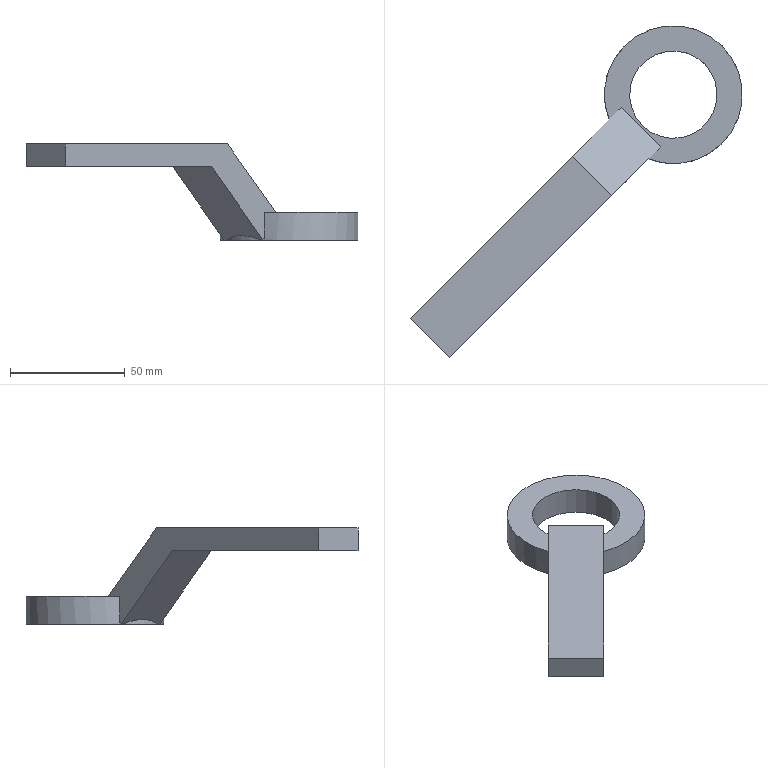Component | NX | WRENCH | 1 solid | 14 faces | box 144.55 x 144.55 x 41.82 mm | volume 56359 mm3 | plane 11 | cylinder 3 | commonest cylinder face diameters 60 x2 38 x1
STEP:
#1=CARTESIAN_POINT('',(0.,0.,0.));
#2=DIRECTION('',(0.,0.,1.));
#3=DIRECTION('',(1.,0.,0.));
#4=AXIS2_PLACEMENT_3D('',#1,#2,#3);
#5=CARTESIAN_POINT('',(53.835,-128.832,-32.615));
#6=VERTEX_POINT('',#5);
#7=CARTESIAN_POINT('',(69.066,-144.064,-32.615));
#8=VERTEX_POINT('',#7);
#9=CARTESIAN_POINT('',(81.249,-116.649,-32.615));
#10=DIRECTION('',(0.,0.,1.));
#11=DIRECTION('',(-0.7071,-0.7071,0.));
#12=AXIS2_PLACEMENT_3D('',#9,#10,#11);
#13=CIRCLE('',#12,30.);
#14=CARTESIAN_POINT('',(81.249,-116.649,-32.615));
#15=DIRECTION('',(0.,0.,1.));
#16=DIRECTION('',(-0.7071,-0.7071,0.));
#17=AXIS2_PLACEMENT_3D('',#14,#15,#16);
#18=CYLINDRICAL_SURFACE('',#17,30.);
#19=CARTESIAN_POINT('',(0.,0.));
#20=DIRECTION('',(1.,0.));
#21=VECTOR('',#20,1.);
#22=LINE('',#19,#21);
#23=(GEOMETRIC_REPRESENTATION_CONTEXT(2)PARAMETRIC_REPRESENTATION_CONTEXT()REPRESENTATION_CONTEXT('',''));
#24=DEFINITIONAL_REPRESENTATION('',(#22),#23);
#25=PCURVE('',#18,#24);
#26=CARTESIAN_POINT('',(81.249,-116.649,-32.615));
#27=DIRECTION('',(0.,0.,-1.));
#28=DIRECTION('',(0.7071,0.7071,0.));
#29=AXIS2_PLACEMENT_3D('',#26,#27,#28);
#30=PLANE('',#29);
#31=CARTESIAN_POINT('',(-30.,0.));
#32=CARTESIAN_POINT('',(-30.,51.962));
#33=CARTESIAN_POINT('',(15.,25.981));
#34=CARTESIAN_POINT('',(60.,0.));
#35=CARTESIAN_POINT('',(15.,-25.981));
#36=CARTESIAN_POINT('',(-30.,-51.962));
#37=CARTESIAN_POINT('',(-30.,0.));
#38=(BOUNDED_CURVE()B_SPLINE_CURVE(2,(#31,#32,#33,#34,#35,#36,#37),.UNSPECIFIED.,.T.,.F.)B_SPLINE_CURVE_WITH_KNOTS((1,2,2,2,2,1),(-2.094,0.,2.094,4.189,6.283,8.378),.UNSPECIFIED.)CURVE()GEOMETRIC_REPRESENTATION_ITEM()RATIONAL_B_SPLINE_CURVE((1.,0.5,1.,0.5,1.,0.5,1.))REPRESENTATION_ITEM(''));
#39=(GEOMETRIC_REPRESENTATION_CONTEXT(2)PARAMETRIC_REPRESENTATION_CONTEXT()REPRESENTATION_CONTEXT('',''));
#40=DEFINITIONAL_REPRESENTATION('',(#38),#39);
#41=PCURVE('',#30,#40);
#42=SURFACE_CURVE('',#13,(#25,#41),.PCURVE_S1.);
#43=EDGE_CURVE('',#6,#8,#42,.T.);
#44=ORIENTED_EDGE('',*,*,#43,.T.);
#45=CARTESIAN_POINT('',(81.249,-116.649,-60.615));
#46=DIRECTION('',(-0.5,-0.5,-0.7071));
#47=DIRECTION('',(-0.5,-0.5,0.7071));
#48=AXIS2_PLACEMENT_3D('',#45,#46,#47);
#49=ELLIPSE('',#48,42.426,30.);
#50=CARTESIAN_POINT('',(6.65,-0.));
#51=CARTESIAN_POINT('',(6.639,0.1198));
#52=CARTESIAN_POINT('',(6.617,0.3491));
#53=CARTESIAN_POINT('',(6.584,0.6615));
#54=CARTESIAN_POINT('',(6.55,0.9419));
#55=CARTESIAN_POINT('',(6.517,1.19));
#56=CARTESIAN_POINT('',(6.483,1.406));
#57=CARTESIAN_POINT('',(6.45,1.589));
#58=CARTESIAN_POINT('',(6.417,1.738));
#59=CARTESIAN_POINT('',(6.383,1.855));
#60=CARTESIAN_POINT('',(6.35,1.939));
#61=CARTESIAN_POINT('',(6.317,1.989));
#62=CARTESIAN_POINT('',(6.283,2.006));
#63=CARTESIAN_POINT('',(6.25,1.989));
#64=CARTESIAN_POINT('',(6.216,1.939));
#65=CARTESIAN_POINT('',(6.183,1.855));
#66=CARTESIAN_POINT('',(6.15,1.738));
#67=CARTESIAN_POINT('',(6.116,1.589));
#68=CARTESIAN_POINT('',(6.083,1.406));
#69=CARTESIAN_POINT('',(6.05,1.19));
#70=CARTESIAN_POINT('',(6.016,0.9419));
#71=CARTESIAN_POINT('',(5.983,0.6615));
#72=CARTESIAN_POINT('',(5.949,0.3491));
#73=CARTESIAN_POINT('',(5.927,0.1198));
#74=CARTESIAN_POINT('',(5.916,-0.));
#75=B_SPLINE_CURVE_WITH_KNOTS('',3,(#50,#51,#52,#53,#54,#55,#56,#57,#58,#59,#60,#61,#62,#63,#64,#65,#66,#67,#68,#69,#70,#71,#72,#73,#74),.UNSPECIFIED.,.F.,.F.,(4,1,1,1,1,1,1,1,1,1,1,1,1,1,1,1,1,1,1,1,1,1,4),(5.916,5.949,5.983,6.016,6.05,6.083,6.116,6.15,6.183,6.216,6.25,6.283,6.317,6.35,6.383,6.417,6.45,6.483,6.517,6.55,6.584,6.617,6.65),.QUASI_UNIFORM_KNOTS.);
#76=(GEOMETRIC_REPRESENTATION_CONTEXT(2)PARAMETRIC_REPRESENTATION_CONTEXT()REPRESENTATION_CONTEXT('',''));
#77=DEFINITIONAL_REPRESENTATION('',(#75),#76);
#78=PCURVE('',#18,#77);
#79=CARTESIAN_POINT('',(52.965,-127.963,-32.615));
#80=DIRECTION('',(0.5,0.5,0.7071));
#81=DIRECTION('',(-0.5,-0.5,0.7071));
#82=AXIS2_PLACEMENT_3D('',#79,#80,#81);
#83=PLANE('',#82);
#84=CARTESIAN_POINT('',(2.828,12.));
#85=CARTESIAN_POINT('',(2.828,-39.962));
#86=CARTESIAN_POINT('',(-60.811,-13.981));
#87=CARTESIAN_POINT('',(-124.451,12.));
#88=CARTESIAN_POINT('',(-60.811,37.981));
#89=CARTESIAN_POINT('',(2.828,63.962));
#90=CARTESIAN_POINT('',(2.828,12.));
#91=(BOUNDED_CURVE()B_SPLINE_CURVE(2,(#84,#85,#86,#87,#88,#89,#90),.UNSPECIFIED.,.T.,.F.)B_SPLINE_CURVE_WITH_KNOTS((1,2,2,2,2,1),(-2.094,0.,2.094,4.189,6.283,8.378),.UNSPECIFIED.)CURVE()GEOMETRIC_REPRESENTATION_ITEM()RATIONAL_B_SPLINE_CURVE((1.,0.5,1.,0.5,1.,0.5,1.))REPRESENTATION_ITEM(''));
#92=(GEOMETRIC_REPRESENTATION_CONTEXT(2)PARAMETRIC_REPRESENTATION_CONTEXT()REPRESENTATION_CONTEXT('',''));
#93=DEFINITIONAL_REPRESENTATION('',(#91),#92);
#94=PCURVE('',#83,#93);
#95=SURFACE_CURVE('',#49,(#78,#94),.PCURVE_S1.);
#96=EDGE_CURVE('',#8,#6,#95,.T.);
#97=ORIENTED_EDGE('',*,*,#96,.T.);
#98=EDGE_LOOP('',(#44,#97));
#99=FACE_BOUND('',#98,.T.);
#100=ADVANCED_FACE('',(#99),#18,.T.);
#101=CARTESIAN_POINT('',(58.494,-122.434,-20.615));
#102=VERTEX_POINT('',#101);
#103=CARTESIAN_POINT('',(53.322,-127.606,-20.615));
#104=VERTEX_POINT('',#103);
#105=CARTESIAN_POINT('',(72.764,-108.164,-20.615));
#106=DIRECTION('',(-0.7071,-0.7071,0.));
#107=VECTOR('',#106,1.);
#108=LINE('',#105,#107);
#109=CARTESIAN_POINT('',(81.249,-116.649,-20.615));
#110=DIRECTION('',(0.,0.,1.));
#111=DIRECTION('',(-0.7071,-0.7071,0.));
#112=AXIS2_PLACEMENT_3D('',#109,#110,#111);
#113=PLANE('',#112);
#114=CARTESIAN_POINT('',(-0.,-12.));
#115=DIRECTION('',(1.,0.));
#116=VECTOR('',#115,1.);
#117=LINE('',#114,#116);
#118=(GEOMETRIC_REPRESENTATION_CONTEXT(2)PARAMETRIC_REPRESENTATION_CONTEXT()REPRESENTATION_CONTEXT('',''));
#119=DEFINITIONAL_REPRESENTATION('',(#117),#118);
#120=PCURVE('',#113,#119);
#121=CARTESIAN_POINT('',(72.764,-108.164,-32.615));
#122=DIRECTION('',(-0.7071,0.7071,0.));
#123=DIRECTION('',(0.,0.,-1.));
#124=AXIS2_PLACEMENT_3D('',#121,#122,#123);
#125=PLANE('',#124);
#126=CARTESIAN_POINT('',(-12.,0.));
#127=DIRECTION('',(0.,1.));
#128=VECTOR('',#127,1.);
#129=LINE('',#126,#128);
#130=(GEOMETRIC_REPRESENTATION_CONTEXT(2)PARAMETRIC_REPRESENTATION_CONTEXT()REPRESENTATION_CONTEXT('',''));
#131=DEFINITIONAL_REPRESENTATION('',(#129),#130);
#132=PCURVE('',#125,#131);
#133=SURFACE_CURVE('',#108,(#120,#132),.PCURVE_S1.);
#134=EDGE_CURVE('',#102,#104,#133,.T.);
#135=ORIENTED_EDGE('',*,*,#134,.F.);
#136=CARTESIAN_POINT('',(75.465,-139.404,-20.615));
#137=VERTEX_POINT('',#136);
#138=CARTESIAN_POINT('',(58.494,-122.434,-20.615));
#139=DIRECTION('',(0.7071,-0.7071,0.));
#140=VECTOR('',#139,1.);
#141=LINE('',#138,#140);
#142=CARTESIAN_POINT('',(20.18,-12.));
#143=DIRECTION('',(0.,1.));
#144=VECTOR('',#143,1.);
#145=LINE('',#142,#144);
#146=(GEOMETRIC_REPRESENTATION_CONTEXT(2)PARAMETRIC_REPRESENTATION_CONTEXT()REPRESENTATION_CONTEXT('',''));
#147=DEFINITIONAL_REPRESENTATION('',(#145),#146);
#148=PCURVE('',#113,#147);
#149=CARTESIAN_POINT('',(37.409,-143.519,9.205));
#150=DIRECTION('',(-0.5,-0.5,-0.7071));
#151=DIRECTION('',(0.5,0.5,-0.7071));
#152=AXIS2_PLACEMENT_3D('',#149,#150,#151);
#153=PLANE('',#152);
#154=CARTESIAN_POINT('',(42.172,0.));
#155=DIRECTION('',(-0.,1.));
#156=VECTOR('',#155,1.);
#157=LINE('',#154,#156);
#158=(GEOMETRIC_REPRESENTATION_CONTEXT(2)PARAMETRIC_REPRESENTATION_CONTEXT()REPRESENTATION_CONTEXT('',''));
#159=DEFINITIONAL_REPRESENTATION('',(#157),#158);
#160=PCURVE('',#153,#159);
#161=SURFACE_CURVE('',#141,(#148,#160),.PCURVE_S1.);
#162=EDGE_CURVE('',#102,#137,#161,.T.);
#163=ORIENTED_EDGE('',*,*,#162,.T.);
#164=CARTESIAN_POINT('',(70.292,-144.577,-20.615));
#165=VERTEX_POINT('',#164);
#166=CARTESIAN_POINT('',(89.735,-125.135,-20.615));
#167=DIRECTION('',(-0.7071,-0.7071,0.));
#168=VECTOR('',#167,1.);
#169=LINE('',#166,#168);
#170=CARTESIAN_POINT('',(-0.,12.));
#171=DIRECTION('',(1.,0.));
#172=VECTOR('',#171,1.);
#173=LINE('',#170,#172);
#174=(GEOMETRIC_REPRESENTATION_CONTEXT(2)PARAMETRIC_REPRESENTATION_CONTEXT()REPRESENTATION_CONTEXT('',''));
#175=DEFINITIONAL_REPRESENTATION('',(#173),#174);
#176=PCURVE('',#113,#175);
#177=CARTESIAN_POINT('',(89.735,-125.135,-32.615));
#178=DIRECTION('',(-0.7071,0.7071,0.));
#179=DIRECTION('',(0.,0.,-1.));
#180=AXIS2_PLACEMENT_3D('',#177,#178,#179);
#181=PLANE('',#180);
#182=CARTESIAN_POINT('',(-12.,0.));
#183=DIRECTION('',(0.,1.));
#184=VECTOR('',#183,1.);
#185=LINE('',#182,#184);
#186=(GEOMETRIC_REPRESENTATION_CONTEXT(2)PARAMETRIC_REPRESENTATION_CONTEXT()REPRESENTATION_CONTEXT('',''));
#187=DEFINITIONAL_REPRESENTATION('',(#185),#186);
#188=PCURVE('',#181,#187);
#189=SURFACE_CURVE('',#169,(#176,#188),.PCURVE_S1.);
#190=EDGE_CURVE('',#137,#165,#189,.T.);
#191=ORIENTED_EDGE('',*,*,#190,.T.);
#192=CARTESIAN_POINT('',(81.249,-116.649,-20.615));
#193=DIRECTION('',(0.,0.,-1.));
#194=DIRECTION('',(-0.7071,-0.7071,0.));
#195=AXIS2_PLACEMENT_3D('',#192,#193,#194);
#196=CIRCLE('',#195,30.);
#197=CARTESIAN_POINT('',(30.,0.));
#198=CARTESIAN_POINT('',(30.,-51.962));
#199=CARTESIAN_POINT('',(-15.,-25.981));
#200=CARTESIAN_POINT('',(-60.,-0.));
#201=CARTESIAN_POINT('',(-15.,25.981));
#202=CARTESIAN_POINT('',(30.,51.962));
#203=CARTESIAN_POINT('',(30.,0.));
#204=(BOUNDED_CURVE()B_SPLINE_CURVE(2,(#197,#198,#199,#200,#201,#202,#203),.UNSPECIFIED.,.T.,.F.)B_SPLINE_CURVE_WITH_KNOTS((1,2,2,2,2,1),(-2.094,0.,2.094,4.189,6.283,8.378),.UNSPECIFIED.)CURVE()GEOMETRIC_REPRESENTATION_ITEM()RATIONAL_B_SPLINE_CURVE((1.,0.5,1.,0.5,1.,0.5,1.))REPRESENTATION_ITEM(''));
#205=(GEOMETRIC_REPRESENTATION_CONTEXT(2)PARAMETRIC_REPRESENTATION_CONTEXT()REPRESENTATION_CONTEXT('',''));
#206=DEFINITIONAL_REPRESENTATION('',(#204),#205);
#207=PCURVE('',#113,#206);
#208=CARTESIAN_POINT('',(81.249,-116.649,-32.615));
#209=DIRECTION('',(0.,0.,1.));
#210=DIRECTION('',(-0.7071,-0.7071,0.));
#211=AXIS2_PLACEMENT_3D('',#208,#209,#210);
#212=CYLINDRICAL_SURFACE('',#211,30.);
#213=CARTESIAN_POINT('',(6.283,12.));
#214=DIRECTION('',(-1.,0.));
#215=VECTOR('',#214,1.);
#216=LINE('',#213,#215);
#217=(GEOMETRIC_REPRESENTATION_CONTEXT(2)PARAMETRIC_REPRESENTATION_CONTEXT()REPRESENTATION_CONTEXT('',''));
#218=DEFINITIONAL_REPRESENTATION('',(#216),#217);
#219=PCURVE('',#212,#218);
#220=SURFACE_CURVE('',#196,(#207,#219),.PCURVE_S1.);
#221=EDGE_CURVE('',#104,#165,#220,.T.);
#222=ORIENTED_EDGE('',*,*,#221,.F.);
#223=EDGE_LOOP('',(#135,#163,#191,#222));
#224=FACE_BOUND('',#223,.T.);
#225=CARTESIAN_POINT('',(67.814,-130.084,-20.615));
#226=VERTEX_POINT('',#225);
#227=CARTESIAN_POINT('',(81.249,-116.649,-20.615));
#228=DIRECTION('',(0.,0.,-1.));
#229=DIRECTION('',(-0.7071,-0.7071,0.));
#230=AXIS2_PLACEMENT_3D('',#227,#228,#229);
#231=CIRCLE('',#230,19.);
#232=CARTESIAN_POINT('',(19.,0.));
#233=CARTESIAN_POINT('',(19.,-32.909));
#234=CARTESIAN_POINT('',(-9.5,-16.454));
#235=CARTESIAN_POINT('',(-38.,-0.));
#236=CARTESIAN_POINT('',(-9.5,16.454));
#237=CARTESIAN_POINT('',(19.,32.909));
#238=CARTESIAN_POINT('',(19.,0.));
#239=(BOUNDED_CURVE()B_SPLINE_CURVE(2,(#232,#233,#234,#235,#236,#237,#238),.UNSPECIFIED.,.T.,.F.)B_SPLINE_CURVE_WITH_KNOTS((1,2,2,2,2,1),(-2.094,0.,2.094,4.189,6.283,8.378),.UNSPECIFIED.)CURVE()GEOMETRIC_REPRESENTATION_ITEM()RATIONAL_B_SPLINE_CURVE((1.,0.5,1.,0.5,1.,0.5,1.))REPRESENTATION_ITEM(''));
#240=(GEOMETRIC_REPRESENTATION_CONTEXT(2)PARAMETRIC_REPRESENTATION_CONTEXT()REPRESENTATION_CONTEXT('',''));
#241=DEFINITIONAL_REPRESENTATION('',(#239),#240);
#242=PCURVE('',#113,#241);
#243=CARTESIAN_POINT('',(81.249,-116.649,-40.615));
#244=DIRECTION('',(0.,0.,1.));
#245=DIRECTION('',(-0.7071,-0.7071,0.));
#246=AXIS2_PLACEMENT_3D('',#243,#244,#245);
#247=CYLINDRICAL_SURFACE('',#246,19.);
#248=CARTESIAN_POINT('',(6.283,20.));
#249=DIRECTION('',(-1.,0.));
#250=VECTOR('',#249,1.);
#251=LINE('',#248,#250);
#252=(GEOMETRIC_REPRESENTATION_CONTEXT(2)PARAMETRIC_REPRESENTATION_CONTEXT()REPRESENTATION_CONTEXT('',''));
#253=DEFINITIONAL_REPRESENTATION('',(#251),#252);
#254=PCURVE('',#247,#253);
#255=SURFACE_CURVE('',#231,(#242,#254),.PCURVE_S1.);
#256=EDGE_CURVE('',#226,#226,#255,.T.);
#257=ORIENTED_EDGE('',*,*,#256,.T.);
#258=EDGE_LOOP('',(#257));
#259=FACE_BOUND('',#258,.T.);
#260=ADVANCED_FACE('',(#224,#259),#113,.T.);
#261=CARTESIAN_POINT('',(81.249,-116.649,-32.615));
#262=DIRECTION('',(0.,0.,1.));
#263=DIRECTION('',(-0.7071,-0.7071,0.));
#264=AXIS2_PLACEMENT_3D('',#261,#262,#263);
#265=CIRCLE('',#264,30.);
#266=CARTESIAN_POINT('',(-30.,0.));
#267=CARTESIAN_POINT('',(-30.,51.962));
#268=CARTESIAN_POINT('',(15.,25.981));
#269=CARTESIAN_POINT('',(60.,0.));
#270=CARTESIAN_POINT('',(15.,-25.981));
#271=CARTESIAN_POINT('',(-30.,-51.962));
#272=CARTESIAN_POINT('',(-30.,0.));
#273=(BOUNDED_CURVE()B_SPLINE_CURVE(2,(#266,#267,#268,#269,#270,#271,#272),.UNSPECIFIED.,.T.,.F.)B_SPLINE_CURVE_WITH_KNOTS((1,2,2,2,2,1),(-2.094,0.,2.094,4.189,6.283,8.378),.UNSPECIFIED.)CURVE()GEOMETRIC_REPRESENTATION_ITEM()RATIONAL_B_SPLINE_CURVE((1.,0.5,1.,0.5,1.,0.5,1.))REPRESENTATION_ITEM(''));
#274=(GEOMETRIC_REPRESENTATION_CONTEXT(2)PARAMETRIC_REPRESENTATION_CONTEXT()REPRESENTATION_CONTEXT('',''));
#275=DEFINITIONAL_REPRESENTATION('',(#273),#274);
#276=PCURVE('',#30,#275);
#277=CARTESIAN_POINT('',(0.,0.));
#278=DIRECTION('',(1.,0.));
#279=VECTOR('',#278,1.);
#280=LINE('',#277,#279);
#281=(GEOMETRIC_REPRESENTATION_CONTEXT(2)PARAMETRIC_REPRESENTATION_CONTEXT()REPRESENTATION_CONTEXT('',''));
#282=DEFINITIONAL_REPRESENTATION('',(#280),#281);
#283=PCURVE('',#212,#282);
#284=SURFACE_CURVE('',#265,(#276,#283),.PCURVE_S1.);
#285=EDGE_CURVE('',#8,#6,#284,.T.);
#286=ORIENTED_EDGE('',*,*,#285,.F.);
#287=ORIENTED_EDGE('',*,*,#43,.F.);
#288=EDGE_LOOP('',(#286,#287));
#289=FACE_BOUND('',#288,.T.);
#290=CARTESIAN_POINT('',(94.684,-103.214,-32.615));
#291=VERTEX_POINT('',#290);
#292=CARTESIAN_POINT('',(67.814,-130.084,-32.615));
#293=VERTEX_POINT('',#292);
#294=CARTESIAN_POINT('',(81.249,-116.649,-32.615));
#295=DIRECTION('',(0.,0.,1.));
#296=DIRECTION('',(0.7071,0.7071,0.));
#297=AXIS2_PLACEMENT_3D('',#294,#295,#296);
#298=CIRCLE('',#297,19.);
#299=CARTESIAN_POINT('',(19.,0.));
#300=CARTESIAN_POINT('',(19.,-32.909));
#301=CARTESIAN_POINT('',(-9.5,-16.454));
#302=CARTESIAN_POINT('',(-38.,-0.));
#303=CARTESIAN_POINT('',(-9.5,16.454));
#304=CARTESIAN_POINT('',(19.,32.909));
#305=CARTESIAN_POINT('',(19.,0.));
#306=(BOUNDED_CURVE()B_SPLINE_CURVE(2,(#299,#300,#301,#302,#303,#304,#305),.UNSPECIFIED.,.T.,.F.)B_SPLINE_CURVE_WITH_KNOTS((1,2,2,2,2,1),(-2.094,0.,2.094,4.189,6.283,8.378),.UNSPECIFIED.)CURVE()GEOMETRIC_REPRESENTATION_ITEM()RATIONAL_B_SPLINE_CURVE((1.,0.5,1.,0.5,1.,0.5,1.))REPRESENTATION_ITEM(''));
#307=(GEOMETRIC_REPRESENTATION_CONTEXT(2)PARAMETRIC_REPRESENTATION_CONTEXT()REPRESENTATION_CONTEXT('',''));
#308=DEFINITIONAL_REPRESENTATION('',(#306),#307);
#309=PCURVE('',#30,#308);
#310=CARTESIAN_POINT('',(3.142,8.));
#311=DIRECTION('',(1.,0.));
#312=VECTOR('',#311,1.);
#313=LINE('',#310,#312);
#314=(GEOMETRIC_REPRESENTATION_CONTEXT(2)PARAMETRIC_REPRESENTATION_CONTEXT()REPRESENTATION_CONTEXT('',''));
#315=DEFINITIONAL_REPRESENTATION('',(#313),#314);
#316=PCURVE('',#247,#315);
#317=SURFACE_CURVE('',#298,(#309,#316),.PCURVE_S1.);
#318=EDGE_CURVE('',#291,#293,#317,.T.);
#319=ORIENTED_EDGE('',*,*,#318,.T.);
#320=CARTESIAN_POINT('',(81.249,-116.649,-32.615));
#321=DIRECTION('',(0.,0.,1.));
#322=DIRECTION('',(0.7071,0.7071,0.));
#323=AXIS2_PLACEMENT_3D('',#320,#321,#322);
#324=CIRCLE('',#323,19.);
#325=CARTESIAN_POINT('',(19.,0.));
#326=CARTESIAN_POINT('',(19.,-32.909));
#327=CARTESIAN_POINT('',(-9.5,-16.454));
#328=CARTESIAN_POINT('',(-38.,-0.));
#329=CARTESIAN_POINT('',(-9.5,16.454));
#330=CARTESIAN_POINT('',(19.,32.909));
#331=CARTESIAN_POINT('',(19.,0.));
#332=(BOUNDED_CURVE()B_SPLINE_CURVE(2,(#325,#326,#327,#328,#329,#330,#331),.UNSPECIFIED.,.T.,.F.)B_SPLINE_CURVE_WITH_KNOTS((1,2,2,2,2,1),(-2.094,0.,2.094,4.189,6.283,8.378),.UNSPECIFIED.)CURVE()GEOMETRIC_REPRESENTATION_ITEM()RATIONAL_B_SPLINE_CURVE((1.,0.5,1.,0.5,1.,0.5,1.))REPRESENTATION_ITEM(''));
#333=(GEOMETRIC_REPRESENTATION_CONTEXT(2)PARAMETRIC_REPRESENTATION_CONTEXT()REPRESENTATION_CONTEXT('',''));
#334=DEFINITIONAL_REPRESENTATION('',(#332),#333);
#335=PCURVE('',#30,#334);
#336=CARTESIAN_POINT('',(-3.142,8.));
#337=DIRECTION('',(1.,0.));
#338=VECTOR('',#337,1.);
#339=LINE('',#336,#338);
#340=(GEOMETRIC_REPRESENTATION_CONTEXT(2)PARAMETRIC_REPRESENTATION_CONTEXT()REPRESENTATION_CONTEXT('',''));
#341=DEFINITIONAL_REPRESENTATION('',(#339),#340);
#342=PCURVE('',#247,#341);
#343=SURFACE_CURVE('',#324,(#335,#342),.PCURVE_S1.);
#344=EDGE_CURVE('',#293,#291,#343,.T.);
#345=ORIENTED_EDGE('',*,*,#344,.T.);
#346=EDGE_LOOP('',(#319,#345));
#347=FACE_BOUND('',#346,.T.);
#348=ADVANCED_FACE('',(#289,#347),#30,.T.);
#349=CARTESIAN_POINT('',(53.322,-127.606,-31.841));
#350=VERTEX_POINT('',#349);
#351=CARTESIAN_POINT('',(53.322,-127.606,-32.615));
#352=DIRECTION('',(0.,0.,-1.));
#353=VECTOR('',#352,1.);
#354=LINE('',#351,#353);
#355=CARTESIAN_POINT('',(5.872,0.));
#356=DIRECTION('',(0.,-1.));
#357=VECTOR('',#356,1.);
#358=LINE('',#355,#357);
#359=(GEOMETRIC_REPRESENTATION_CONTEXT(2)PARAMETRIC_REPRESENTATION_CONTEXT()REPRESENTATION_CONTEXT('',''));
#360=DEFINITIONAL_REPRESENTATION('',(#358),#359);
#361=PCURVE('',#212,#360);
#362=CARTESIAN_POINT('',(0.,27.495));
#363=DIRECTION('',(1.,0.));
#364=VECTOR('',#363,1.);
#365=LINE('',#362,#364);
#366=(GEOMETRIC_REPRESENTATION_CONTEXT(2)PARAMETRIC_REPRESENTATION_CONTEXT()REPRESENTATION_CONTEXT('',''));
#367=DEFINITIONAL_REPRESENTATION('',(#365),#366);
#368=PCURVE('',#125,#367);
#369=SURFACE_CURVE('',#354,(#361,#368),.PCURVE_S1.);
#370=EDGE_CURVE('',#104,#350,#369,.T.);
#371=ORIENTED_EDGE('',*,*,#370,.F.);
#372=ORIENTED_EDGE('',*,*,#221,.T.);
#373=CARTESIAN_POINT('',(70.292,-144.577,-31.841));
#374=VERTEX_POINT('',#373);
#375=CARTESIAN_POINT('',(70.292,-144.577,-32.615));
#376=DIRECTION('',(0.,0.,-1.));
#377=VECTOR('',#376,1.);
#378=LINE('',#375,#377);
#379=CARTESIAN_POINT('',(0.4115,0.));
#380=DIRECTION('',(0.,-1.));
#381=VECTOR('',#380,1.);
#382=LINE('',#379,#381);
#383=(GEOMETRIC_REPRESENTATION_CONTEXT(2)PARAMETRIC_REPRESENTATION_CONTEXT()REPRESENTATION_CONTEXT('',''));
#384=DEFINITIONAL_REPRESENTATION('',(#382),#383);
#385=PCURVE('',#212,#384);
#386=CARTESIAN_POINT('',(0.,27.495));
#387=DIRECTION('',(1.,0.));
#388=VECTOR('',#387,1.);
#389=LINE('',#386,#388);
#390=(GEOMETRIC_REPRESENTATION_CONTEXT(2)PARAMETRIC_REPRESENTATION_CONTEXT()REPRESENTATION_CONTEXT('',''));
#391=DEFINITIONAL_REPRESENTATION('',(#389),#390);
#392=PCURVE('',#181,#391);
#393=SURFACE_CURVE('',#378,(#385,#392),.PCURVE_S1.);
#394=EDGE_CURVE('',#165,#374,#393,.T.);
#395=ORIENTED_EDGE('',*,*,#394,.T.);
#396=CARTESIAN_POINT('',(81.249,-116.649,10.353));
#397=DIRECTION('',(0.5924,0.5924,-0.546));
#398=DIRECTION('',(0.3861,0.3861,0.8378));
#399=AXIS2_PLACEMENT_3D('',#396,#397,#398);
#400=ELLIPSE('',#399,54.949,30.);
#401=CARTESIAN_POINT('',(0.4115,0.7743));
#402=CARTESIAN_POINT('',(0.3672,-0.));
#403=B_SPLINE_CURVE_WITH_KNOTS('',1,(#401,#402),.UNSPECIFIED.,.F.,.F.,(2,2),(2.73,2.774),.PIECEWISE_BEZIER_KNOTS.);
#404=(GEOMETRIC_REPRESENTATION_CONTEXT(2)PARAMETRIC_REPRESENTATION_CONTEXT()REPRESENTATION_CONTEXT('',''));
#405=DEFINITIONAL_REPRESENTATION('',(#403),#404);
#406=PCURVE('',#212,#405);
#407=CARTESIAN_POINT('',(58.494,-122.434,-20.615));
#408=DIRECTION('',(-0.5924,-0.5924,0.546));
#409=DIRECTION('',(-0.3861,-0.3861,-0.8378));
#410=AXIS2_PLACEMENT_3D('',#407,#408,#409);
#411=PLANE('',#410);
#412=CARTESIAN_POINT('',(-91.912,12.));
#413=CARTESIAN_POINT('',(-91.912,63.962));
#414=CARTESIAN_POINT('',(-9.488,37.981));
#415=CARTESIAN_POINT('',(72.935,12.));
#416=CARTESIAN_POINT('',(-9.488,-13.981));
#417=CARTESIAN_POINT('',(-91.912,-39.962));
#418=CARTESIAN_POINT('',(-91.912,12.));
#419=(BOUNDED_CURVE()B_SPLINE_CURVE(2,(#412,#413,#414,#415,#416,#417,#418),.UNSPECIFIED.,.T.,.F.)B_SPLINE_CURVE_WITH_KNOTS((1,2,2,2,2,1),(-2.094,0.,2.094,4.189,6.283,8.378),.UNSPECIFIED.)CURVE()GEOMETRIC_REPRESENTATION_ITEM()RATIONAL_B_SPLINE_CURVE((1.,0.5,1.,0.5,1.,0.5,1.))REPRESENTATION_ITEM(''));
#420=(GEOMETRIC_REPRESENTATION_CONTEXT(2)PARAMETRIC_REPRESENTATION_CONTEXT()REPRESENTATION_CONTEXT('',''));
#421=DEFINITIONAL_REPRESENTATION('',(#419),#420);
#422=PCURVE('',#411,#421);
#423=SURFACE_CURVE('',#400,(#406,#422),.PCURVE_S1.);
#424=EDGE_CURVE('',#374,#8,#423,.T.);
#425=ORIENTED_EDGE('',*,*,#424,.T.);
#426=ORIENTED_EDGE('',*,*,#285,.T.);
#427=CARTESIAN_POINT('',(81.249,-116.649,10.353));
#428=DIRECTION('',(0.5924,0.5924,-0.546));
#429=DIRECTION('',(0.3861,0.3861,0.8378));
#430=AXIS2_PLACEMENT_3D('',#427,#428,#429);
#431=ELLIPSE('',#430,54.949,30.);
#432=CARTESIAN_POINT('',(5.916,0.));
#433=CARTESIAN_POINT('',(5.872,0.7743));
#434=B_SPLINE_CURVE_WITH_KNOTS('',1,(#432,#433),.UNSPECIFIED.,.F.,.F.,(2,2),(3.509,3.553),.PIECEWISE_BEZIER_KNOTS.);
#435=(GEOMETRIC_REPRESENTATION_CONTEXT(2)PARAMETRIC_REPRESENTATION_CONTEXT()REPRESENTATION_CONTEXT('',''));
#436=DEFINITIONAL_REPRESENTATION('',(#434),#435);
#437=PCURVE('',#212,#436);
#438=CARTESIAN_POINT('',(58.494,-122.434,-20.615));
#439=DIRECTION('',(-0.5924,-0.5924,0.546));
#440=DIRECTION('',(-0.3861,-0.3861,-0.8378));
#441=AXIS2_PLACEMENT_3D('',#438,#439,#440);
#442=PLANE('',#441);
#443=CARTESIAN_POINT('',(-91.912,12.));
#444=CARTESIAN_POINT('',(-91.912,63.962));
#445=CARTESIAN_POINT('',(-9.488,37.981));
#446=CARTESIAN_POINT('',(72.935,12.));
#447=CARTESIAN_POINT('',(-9.488,-13.981));
#448=CARTESIAN_POINT('',(-91.912,-39.962));
#449=CARTESIAN_POINT('',(-91.912,12.));
#450=(BOUNDED_CURVE()B_SPLINE_CURVE(2,(#443,#444,#445,#446,#447,#448,#449),.UNSPECIFIED.,.T.,.F.)B_SPLINE_CURVE_WITH_KNOTS((1,2,2,2,2,1),(-2.094,0.,2.094,4.189,6.283,8.378),.UNSPECIFIED.)CURVE()GEOMETRIC_REPRESENTATION_ITEM()RATIONAL_B_SPLINE_CURVE((1.,0.5,1.,0.5,1.,0.5,1.))REPRESENTATION_ITEM(''));
#451=(GEOMETRIC_REPRESENTATION_CONTEXT(2)PARAMETRIC_REPRESENTATION_CONTEXT()REPRESENTATION_CONTEXT('',''));
#452=DEFINITIONAL_REPRESENTATION('',(#450),#451);
#453=PCURVE('',#442,#452);
#454=SURFACE_CURVE('',#431,(#437,#453),.PCURVE_S1.);
#455=EDGE_CURVE('',#6,#350,#454,.T.);
#456=ORIENTED_EDGE('',*,*,#455,.T.);
#457=EDGE_LOOP('',(#371,#372,#395,#425,#426,#456));
#458=FACE_BOUND('',#457,.T.);
#459=ADVANCED_FACE('',(#458),#212,.T.);
#460=ORIENTED_EDGE('',*,*,#318,.T.);
#461=CARTESIAN_POINT('',(67.814,-130.084,-32.615));
#462=CARTESIAN_POINT('',(67.814,-130.084,-20.615));
#463=B_SPLINE_CURVE_WITH_KNOTS('',1,(#461,#462),.UNSPECIFIED.,.F.,.F.,(2,2),(8.,20.),.PIECEWISE_BEZIER_KNOTS.);
#464=CARTESIAN_POINT('',(6.283,0.));
#465=DIRECTION('',(0.,1.));
#466=VECTOR('',#465,1.);
#467=LINE('',#464,#466);
#468=(GEOMETRIC_REPRESENTATION_CONTEXT(2)PARAMETRIC_REPRESENTATION_CONTEXT()REPRESENTATION_CONTEXT('',''));
#469=DEFINITIONAL_REPRESENTATION('',(#467),#468);
#470=PCURVE('',#247,#469);
#471=CARTESIAN_POINT('',(0.,0.));
#472=DIRECTION('',(0.,1.));
#473=VECTOR('',#472,1.);
#474=LINE('',#471,#473);
#475=(GEOMETRIC_REPRESENTATION_CONTEXT(2)PARAMETRIC_REPRESENTATION_CONTEXT()REPRESENTATION_CONTEXT('',''));
#476=DEFINITIONAL_REPRESENTATION('',(#474),#475);
#477=PCURVE('',#247,#476);
#478=SEAM_CURVE('',#463,(#470,#477),.PCURVE_S1.);
#479=EDGE_CURVE('',#293,#226,#478,.T.);
#480=ORIENTED_EDGE('',*,*,#479,.T.);
#481=ORIENTED_EDGE('',*,*,#256,.T.);
#482=ORIENTED_EDGE('',*,*,#479,.F.);
#483=ORIENTED_EDGE('',*,*,#344,.T.);
#484=EDGE_LOOP('',(#460,#480,#481,#482,#483));
#485=FACE_BOUND('',#484,.F.);
#486=ADVANCED_FACE('',(#485),#247,.F.);
#487=ORIENTED_EDGE('',*,*,#424,.F.);
#488=CARTESIAN_POINT('',(69.936,-144.934,-32.615));
#489=VERTEX_POINT('',#488);
#490=CARTESIAN_POINT('',(75.465,-139.404,-20.615));
#491=DIRECTION('',(-0.3861,-0.3861,-0.8378));
#492=VECTOR('',#491,1.);
#493=LINE('',#490,#492);
#494=CARTESIAN_POINT('',(-0.,24.));
#495=DIRECTION('',(1.,0.));
#496=VECTOR('',#495,1.);
#497=LINE('',#494,#496);
#498=(GEOMETRIC_REPRESENTATION_CONTEXT(2)PARAMETRIC_REPRESENTATION_CONTEXT()REPRESENTATION_CONTEXT('',''));
#499=DEFINITIONAL_REPRESENTATION('',(#497),#498);
#500=PCURVE('',#411,#499);
#501=CARTESIAN_POINT('',(-12.,20.18));
#502=DIRECTION('',(0.8378,0.546));
#503=VECTOR('',#502,1.);
#504=LINE('',#501,#503);
#505=(GEOMETRIC_REPRESENTATION_CONTEXT(2)PARAMETRIC_REPRESENTATION_CONTEXT()REPRESENTATION_CONTEXT('',''));
#506=DEFINITIONAL_REPRESENTATION('',(#504),#505);
#507=PCURVE('',#181,#506);
#508=SURFACE_CURVE('',#493,(#500,#507),.PCURVE_S1.);
#509=EDGE_CURVE('',#374,#489,#508,.T.);
#510=ORIENTED_EDGE('',*,*,#509,.T.);
#511=CARTESIAN_POINT('',(52.965,-127.963,-32.615));
#512=DIRECTION('',(0.7071,-0.7071,0.));
#513=VECTOR('',#512,1.);
#514=LINE('',#511,#513);
#515=CARTESIAN_POINT('',(14.323,-0.));
#516=DIRECTION('',(-0.,1.));
#517=VECTOR('',#516,1.);
#518=LINE('',#515,#517);
#519=(GEOMETRIC_REPRESENTATION_CONTEXT(2)PARAMETRIC_REPRESENTATION_CONTEXT()REPRESENTATION_CONTEXT('',''));
#520=DEFINITIONAL_REPRESENTATION('',(#518),#519);
#521=PCURVE('',#411,#520);
#522=CARTESIAN_POINT('',(-0.,0.));
#523=DIRECTION('',(-0.,1.));
#524=VECTOR('',#523,1.);
#525=LINE('',#522,#524);
#526=(GEOMETRIC_REPRESENTATION_CONTEXT(2)PARAMETRIC_REPRESENTATION_CONTEXT()REPRESENTATION_CONTEXT('',''));
#527=DEFINITIONAL_REPRESENTATION('',(#525),#526);
#528=PCURVE('',#83,#527);
#529=SURFACE_CURVE('',#514,(#521,#528),.PCURVE_S1.);
#530=EDGE_CURVE('',#8,#489,#529,.T.);
#531=ORIENTED_EDGE('',*,*,#530,.F.);
#532=EDGE_LOOP('',(#487,#510,#531));
#533=FACE_BOUND('',#532,.T.);
#534=ADVANCED_FACE('',(#533),#411,.F.);
#535=CARTESIAN_POINT('',(54.379,-160.49,9.205));
#536=VERTEX_POINT('',#535);
#537=CARTESIAN_POINT('',(54.379,-160.49,9.205));
#538=DIRECTION('',(0.5,0.5,-0.7071));
#539=VECTOR('',#538,1.);
#540=LINE('',#537,#539);
#541=CARTESIAN_POINT('',(-0.,24.));
#542=DIRECTION('',(1.,0.));
#543=VECTOR('',#542,1.);
#544=LINE('',#541,#543);
#545=(GEOMETRIC_REPRESENTATION_CONTEXT(2)PARAMETRIC_REPRESENTATION_CONTEXT()REPRESENTATION_CONTEXT('',''));
#546=DEFINITIONAL_REPRESENTATION('',(#544),#545);
#547=PCURVE('',#153,#546);
#548=CARTESIAN_POINT('',(-41.82,50.));
#549=DIRECTION('',(0.7071,-0.7071));
#550=VECTOR('',#549,1.);
#551=LINE('',#548,#550);
#552=(GEOMETRIC_REPRESENTATION_CONTEXT(2)PARAMETRIC_REPRESENTATION_CONTEXT()REPRESENTATION_CONTEXT('',''));
#553=DEFINITIONAL_REPRESENTATION('',(#551),#552);
#554=PCURVE('',#181,#553);
#555=SURFACE_CURVE('',#540,(#547,#554),.PCURVE_S1.);
#556=EDGE_CURVE('',#536,#137,#555,.T.);
#557=ORIENTED_EDGE('',*,*,#556,.T.);
#558=ORIENTED_EDGE('',*,*,#162,.F.);
#559=CARTESIAN_POINT('',(37.409,-143.519,9.205));
#560=VERTEX_POINT('',#559);
#561=CARTESIAN_POINT('',(37.409,-143.519,9.205));
#562=DIRECTION('',(0.5,0.5,-0.7071));
#563=VECTOR('',#562,1.);
#564=LINE('',#561,#563);
#565=CARTESIAN_POINT('',(0.,0.));
#566=DIRECTION('',(1.,0.));
#567=VECTOR('',#566,1.);
#568=LINE('',#565,#567);
#569=(GEOMETRIC_REPRESENTATION_CONTEXT(2)PARAMETRIC_REPRESENTATION_CONTEXT()REPRESENTATION_CONTEXT('',''));
#570=DEFINITIONAL_REPRESENTATION('',(#568),#569);
#571=PCURVE('',#153,#570);
#572=CARTESIAN_POINT('',(-41.82,50.));
#573=DIRECTION('',(0.7071,-0.7071));
#574=VECTOR('',#573,1.);
#575=LINE('',#572,#574);
#576=(GEOMETRIC_REPRESENTATION_CONTEXT(2)PARAMETRIC_REPRESENTATION_CONTEXT()REPRESENTATION_CONTEXT('',''));
#577=DEFINITIONAL_REPRESENTATION('',(#575),#576);
#578=PCURVE('',#125,#577);
#579=SURFACE_CURVE('',#564,(#571,#578),.PCURVE_S1.);
#580=EDGE_CURVE('',#560,#102,#579,.T.);
#581=ORIENTED_EDGE('',*,*,#580,.F.);
#582=CARTESIAN_POINT('',(37.409,-143.519,9.205));
#583=DIRECTION('',(0.7071,-0.7071,0.));
#584=VECTOR('',#583,1.);
#585=LINE('',#582,#584);
#586=CARTESIAN_POINT('',(0.,0.));
#587=DIRECTION('',(-0.,1.));
#588=VECTOR('',#587,1.);
#589=LINE('',#586,#588);
#590=(GEOMETRIC_REPRESENTATION_CONTEXT(2)PARAMETRIC_REPRESENTATION_CONTEXT()REPRESENTATION_CONTEXT('',''));
#591=DEFINITIONAL_REPRESENTATION('',(#589),#590);
#592=PCURVE('',#153,#591);
#593=CARTESIAN_POINT('',(-33.302,-214.23,9.205));
#594=DIRECTION('',(0.,0.,-1.));
#595=DIRECTION('',(0.7071,0.7071,0.));
#596=AXIS2_PLACEMENT_3D('',#593,#594,#595);
#597=PLANE('',#596);
#598=CARTESIAN_POINT('',(100.,-0.));
#599=DIRECTION('',(-0.,1.));
#600=VECTOR('',#599,1.);
#601=LINE('',#598,#600);
#602=(GEOMETRIC_REPRESENTATION_CONTEXT(2)PARAMETRIC_REPRESENTATION_CONTEXT()REPRESENTATION_CONTEXT('',''));
#603=DEFINITIONAL_REPRESENTATION('',(#601),#602);
#604=PCURVE('',#597,#603);
#605=SURFACE_CURVE('',#585,(#592,#604),.PCURVE_S1.);
#606=EDGE_CURVE('',#560,#536,#605,.T.);
#607=ORIENTED_EDGE('',*,*,#606,.T.);
#608=EDGE_LOOP('',(#557,#558,#581,#607));
#609=FACE_BOUND('',#608,.T.);
#610=ADVANCED_FACE('',(#609),#153,.F.);
#611=ORIENTED_EDGE('',*,*,#455,.F.);
#612=CARTESIAN_POINT('',(52.965,-127.963,-32.615));
#613=VERTEX_POINT('',#612);
#614=CARTESIAN_POINT('',(52.965,-127.963,-32.615));
#615=DIRECTION('',(0.7071,-0.7071,0.));
#616=VECTOR('',#615,1.);
#617=LINE('',#614,#616);
#618=CARTESIAN_POINT('',(14.323,-0.));
#619=DIRECTION('',(-0.,1.));
#620=VECTOR('',#619,1.);
#621=LINE('',#618,#620);
#622=(GEOMETRIC_REPRESENTATION_CONTEXT(2)PARAMETRIC_REPRESENTATION_CONTEXT()REPRESENTATION_CONTEXT('',''));
#623=DEFINITIONAL_REPRESENTATION('',(#621),#622);
#624=PCURVE('',#442,#623);
#625=CARTESIAN_POINT('',(-0.,0.));
#626=DIRECTION('',(-0.,1.));
#627=VECTOR('',#626,1.);
#628=LINE('',#625,#627);
#629=(GEOMETRIC_REPRESENTATION_CONTEXT(2)PARAMETRIC_REPRESENTATION_CONTEXT()REPRESENTATION_CONTEXT('',''));
#630=DEFINITIONAL_REPRESENTATION('',(#628),#629);
#631=PCURVE('',#83,#630);
#632=SURFACE_CURVE('',#617,(#624,#631),.PCURVE_S1.);
#633=EDGE_CURVE('',#613,#6,#632,.T.);
#634=ORIENTED_EDGE('',*,*,#633,.F.);
#635=CARTESIAN_POINT('',(58.494,-122.434,-20.615));
#636=DIRECTION('',(-0.3861,-0.3861,-0.8378));
#637=VECTOR('',#636,1.);
#638=LINE('',#635,#637);
#639=CARTESIAN_POINT('',(0.,0.));
#640=DIRECTION('',(1.,0.));
#641=VECTOR('',#640,1.);
#642=LINE('',#639,#641);
#643=(GEOMETRIC_REPRESENTATION_CONTEXT(2)PARAMETRIC_REPRESENTATION_CONTEXT()REPRESENTATION_CONTEXT('',''));
#644=DEFINITIONAL_REPRESENTATION('',(#642),#643);
#645=PCURVE('',#442,#644);
#646=CARTESIAN_POINT('',(-12.,20.18));
#647=DIRECTION('',(0.8378,0.546));
#648=VECTOR('',#647,1.);
#649=LINE('',#646,#648);
#650=(GEOMETRIC_REPRESENTATION_CONTEXT(2)PARAMETRIC_REPRESENTATION_CONTEXT()REPRESENTATION_CONTEXT('',''));
#651=DEFINITIONAL_REPRESENTATION('',(#649),#650);
#652=PCURVE('',#125,#651);
#653=SURFACE_CURVE('',#638,(#645,#652),.PCURVE_S1.);
#654=EDGE_CURVE('',#350,#613,#653,.T.);
#655=ORIENTED_EDGE('',*,*,#654,.F.);
#656=EDGE_LOOP('',(#611,#634,#655));
#657=FACE_BOUND('',#656,.T.);
#658=ADVANCED_FACE('',(#657),#442,.F.);
#659=ORIENTED_EDGE('',*,*,#96,.F.);
#660=ORIENTED_EDGE('',*,*,#530,.T.);
#661=CARTESIAN_POINT('',(47.436,-167.434,-0.7954));
#662=VERTEX_POINT('',#661);
#663=CARTESIAN_POINT('',(69.936,-144.934,-32.615));
#664=DIRECTION('',(-0.5,-0.5,0.7071));
#665=VECTOR('',#664,1.);
#666=LINE('',#663,#665);
#667=CARTESIAN_POINT('',(0.,24.));
#668=DIRECTION('',(1.,0.));
#669=VECTOR('',#668,1.);
#670=LINE('',#667,#669);
#671=(GEOMETRIC_REPRESENTATION_CONTEXT(2)PARAMETRIC_REPRESENTATION_CONTEXT()REPRESENTATION_CONTEXT('',''));
#672=DEFINITIONAL_REPRESENTATION('',(#670),#671);
#673=PCURVE('',#83,#672);
#674=CARTESIAN_POINT('',(0.,28.));
#675=DIRECTION('',(-0.7071,0.7071));
#676=VECTOR('',#675,1.);
#677=LINE('',#674,#676);
#678=(GEOMETRIC_REPRESENTATION_CONTEXT(2)PARAMETRIC_REPRESENTATION_CONTEXT()REPRESENTATION_CONTEXT('',''));
#679=DEFINITIONAL_REPRESENTATION('',(#677),#678);
#680=PCURVE('',#181,#679);
#681=SURFACE_CURVE('',#666,(#673,#680),.PCURVE_S1.);
#682=EDGE_CURVE('',#489,#662,#681,.T.);
#683=ORIENTED_EDGE('',*,*,#682,.T.);
#684=CARTESIAN_POINT('',(30.465,-150.463,-0.7954));
#685=VERTEX_POINT('',#684);
#686=CARTESIAN_POINT('',(30.465,-150.463,-0.7954));
#687=DIRECTION('',(0.7071,-0.7071,0.));
#688=VECTOR('',#687,1.);
#689=LINE('',#686,#688);
#690=CARTESIAN_POINT('',(45.,0.));
#691=DIRECTION('',(-0.,1.));
#692=VECTOR('',#691,1.);
#693=LINE('',#690,#692);
#694=(GEOMETRIC_REPRESENTATION_CONTEXT(2)PARAMETRIC_REPRESENTATION_CONTEXT()REPRESENTATION_CONTEXT('',''));
#695=DEFINITIONAL_REPRESENTATION('',(#693),#694);
#696=PCURVE('',#83,#695);
#697=CARTESIAN_POINT('',(30.465,-150.463,-0.7954));
#698=DIRECTION('',(0.,0.,1.));
#699=DIRECTION('',(-0.7071,-0.7071,0.));
#700=AXIS2_PLACEMENT_3D('',#697,#698,#699);
#701=PLANE('',#700);
#702=CARTESIAN_POINT('',(0.,0.));
#703=DIRECTION('',(0.,1.));
#704=VECTOR('',#703,1.);
#705=LINE('',#702,#704);
#706=(GEOMETRIC_REPRESENTATION_CONTEXT(2)PARAMETRIC_REPRESENTATION_CONTEXT()REPRESENTATION_CONTEXT('',''));
#707=DEFINITIONAL_REPRESENTATION('',(#705),#706);
#708=PCURVE('',#701,#707);
#709=SURFACE_CURVE('',#689,(#696,#708),.PCURVE_S1.);
#710=EDGE_CURVE('',#685,#662,#709,.T.);
#711=ORIENTED_EDGE('',*,*,#710,.F.);
#712=CARTESIAN_POINT('',(52.965,-127.963,-32.615));
#713=DIRECTION('',(-0.5,-0.5,0.7071));
#714=VECTOR('',#713,1.);
#715=LINE('',#712,#714);
#716=CARTESIAN_POINT('',(0.,0.));
#717=DIRECTION('',(1.,0.));
#718=VECTOR('',#717,1.);
#719=LINE('',#716,#718);
#720=(GEOMETRIC_REPRESENTATION_CONTEXT(2)PARAMETRIC_REPRESENTATION_CONTEXT()REPRESENTATION_CONTEXT('',''));
#721=DEFINITIONAL_REPRESENTATION('',(#719),#720);
#722=PCURVE('',#83,#721);
#723=CARTESIAN_POINT('',(0.,28.));
#724=DIRECTION('',(-0.7071,0.7071));
#725=VECTOR('',#724,1.);
#726=LINE('',#723,#725);
#727=(GEOMETRIC_REPRESENTATION_CONTEXT(2)PARAMETRIC_REPRESENTATION_CONTEXT()REPRESENTATION_CONTEXT('',''));
#728=DEFINITIONAL_REPRESENTATION('',(#726),#727);
#729=PCURVE('',#125,#728);
#730=SURFACE_CURVE('',#715,(#722,#729),.PCURVE_S1.);
#731=EDGE_CURVE('',#613,#685,#730,.T.);
#732=ORIENTED_EDGE('',*,*,#731,.F.);
#733=ORIENTED_EDGE('',*,*,#633,.T.);
#734=EDGE_LOOP('',(#659,#660,#683,#711,#732,#733));
#735=FACE_BOUND('',#734,.T.);
#736=ADVANCED_FACE('',(#735),#83,.F.);
#737=CARTESIAN_POINT('',(-16.331,-231.201,-0.7954));
#738=VERTEX_POINT('',#737);
#739=CARTESIAN_POINT('',(47.436,-167.434,-0.7954));
#740=DIRECTION('',(-0.7071,-0.7071,0.));
#741=VECTOR('',#740,1.);
#742=LINE('',#739,#741);
#743=CARTESIAN_POINT('',(0.,24.));
#744=DIRECTION('',(1.,0.));
#745=VECTOR('',#744,1.);
#746=LINE('',#743,#745);
#747=(GEOMETRIC_REPRESENTATION_CONTEXT(2)PARAMETRIC_REPRESENTATION_CONTEXT()REPRESENTATION_CONTEXT('',''));
#748=DEFINITIONAL_REPRESENTATION('',(#746),#747);
#749=PCURVE('',#701,#748);
#750=CARTESIAN_POINT('',(-31.82,59.82));
#751=DIRECTION('',(0.,1.));
#752=VECTOR('',#751,1.);
#753=LINE('',#750,#752);
#754=(GEOMETRIC_REPRESENTATION_CONTEXT(2)PARAMETRIC_REPRESENTATION_CONTEXT()REPRESENTATION_CONTEXT('',''));
#755=DEFINITIONAL_REPRESENTATION('',(#753),#754);
#756=PCURVE('',#181,#755);
#757=SURFACE_CURVE('',#742,(#749,#756),.PCURVE_S1.);
#758=EDGE_CURVE('',#662,#738,#757,.T.);
#759=ORIENTED_EDGE('',*,*,#758,.T.);
#760=CARTESIAN_POINT('',(-33.302,-214.23,-0.7954));
#761=VERTEX_POINT('',#760);
#762=CARTESIAN_POINT('',(-33.302,-214.23,-0.7954));
#763=DIRECTION('',(0.7071,-0.7071,0.));
#764=VECTOR('',#763,1.);
#765=LINE('',#762,#764);
#766=CARTESIAN_POINT('',(90.18,0.));
#767=DIRECTION('',(0.,1.));
#768=VECTOR('',#767,1.);
#769=LINE('',#766,#768);
#770=(GEOMETRIC_REPRESENTATION_CONTEXT(2)PARAMETRIC_REPRESENTATION_CONTEXT()REPRESENTATION_CONTEXT('',''));
#771=DEFINITIONAL_REPRESENTATION('',(#769),#770);
#772=PCURVE('',#701,#771);
#773=CARTESIAN_POINT('',(-33.302,-214.23,-0.7954));
#774=DIRECTION('',(0.7071,0.7071,0.));
#775=DIRECTION('',(0.,0.,1.));
#776=AXIS2_PLACEMENT_3D('',#773,#774,#775);
#777=PLANE('',#776);
#778=CARTESIAN_POINT('',(0.,0.));
#779=DIRECTION('',(0.,1.));
#780=VECTOR('',#779,1.);
#781=LINE('',#778,#780);
#782=(GEOMETRIC_REPRESENTATION_CONTEXT(2)PARAMETRIC_REPRESENTATION_CONTEXT()REPRESENTATION_CONTEXT('',''));
#783=DEFINITIONAL_REPRESENTATION('',(#781),#782);
#784=PCURVE('',#777,#783);
#785=SURFACE_CURVE('',#765,(#772,#784),.PCURVE_S1.);
#786=EDGE_CURVE('',#761,#738,#785,.T.);
#787=ORIENTED_EDGE('',*,*,#786,.F.);
#788=CARTESIAN_POINT('',(30.465,-150.463,-0.7954));
#789=DIRECTION('',(-0.7071,-0.7071,0.));
#790=VECTOR('',#789,1.);
#791=LINE('',#788,#790);
#792=CARTESIAN_POINT('',(0.,0.));
#793=DIRECTION('',(1.,0.));
#794=VECTOR('',#793,1.);
#795=LINE('',#792,#794);
#796=(GEOMETRIC_REPRESENTATION_CONTEXT(2)PARAMETRIC_REPRESENTATION_CONTEXT()REPRESENTATION_CONTEXT('',''));
#797=DEFINITIONAL_REPRESENTATION('',(#795),#796);
#798=PCURVE('',#701,#797);
#799=CARTESIAN_POINT('',(-31.82,59.82));
#800=DIRECTION('',(0.,1.));
#801=VECTOR('',#800,1.);
#802=LINE('',#799,#801);
#803=(GEOMETRIC_REPRESENTATION_CONTEXT(2)PARAMETRIC_REPRESENTATION_CONTEXT()REPRESENTATION_CONTEXT('',''));
#804=DEFINITIONAL_REPRESENTATION('',(#802),#803);
#805=PCURVE('',#125,#804);
#806=SURFACE_CURVE('',#791,(#798,#805),.PCURVE_S1.);
#807=EDGE_CURVE('',#685,#761,#806,.T.);
#808=ORIENTED_EDGE('',*,*,#807,.F.);
#809=ORIENTED_EDGE('',*,*,#710,.T.);
#810=EDGE_LOOP('',(#759,#787,#808,#809));
#811=FACE_BOUND('',#810,.T.);
#812=ADVANCED_FACE('',(#811),#701,.F.);
#813=CARTESIAN_POINT('',(-16.331,-231.201,9.205));
#814=VERTEX_POINT('',#813);
#815=CARTESIAN_POINT('',(-16.331,-231.201,-0.7954));
#816=DIRECTION('',(0.,0.,1.));
#817=VECTOR('',#816,1.);
#818=LINE('',#815,#817);
#819=CARTESIAN_POINT('',(0.,24.));
#820=DIRECTION('',(1.,0.));
#821=VECTOR('',#820,1.);
#822=LINE('',#819,#821);
#823=(GEOMETRIC_REPRESENTATION_CONTEXT(2)PARAMETRIC_REPRESENTATION_CONTEXT()REPRESENTATION_CONTEXT('',''));
#824=DEFINITIONAL_REPRESENTATION('',(#822),#823);
#825=PCURVE('',#777,#824);
#826=CARTESIAN_POINT('',(-31.82,150.));
#827=DIRECTION('',(-1.,0.));
#828=VECTOR('',#827,1.);
#829=LINE('',#826,#828);
#830=(GEOMETRIC_REPRESENTATION_CONTEXT(2)PARAMETRIC_REPRESENTATION_CONTEXT()REPRESENTATION_CONTEXT('',''));
#831=DEFINITIONAL_REPRESENTATION('',(#829),#830);
#832=PCURVE('',#181,#831);
#833=SURFACE_CURVE('',#818,(#825,#832),.PCURVE_S1.);
#834=EDGE_CURVE('',#738,#814,#833,.T.);
#835=ORIENTED_EDGE('',*,*,#834,.T.);
#836=CARTESIAN_POINT('',(-33.302,-214.23,9.205));
#837=VERTEX_POINT('',#836);
#838=CARTESIAN_POINT('',(-33.302,-214.23,9.205));
#839=DIRECTION('',(0.7071,-0.7071,0.));
#840=VECTOR('',#839,1.);
#841=LINE('',#838,#840);
#842=CARTESIAN_POINT('',(10.,0.));
#843=DIRECTION('',(0.,1.));
#844=VECTOR('',#843,1.);
#845=LINE('',#842,#844);
#846=(GEOMETRIC_REPRESENTATION_CONTEXT(2)PARAMETRIC_REPRESENTATION_CONTEXT()REPRESENTATION_CONTEXT('',''));
#847=DEFINITIONAL_REPRESENTATION('',(#845),#846);
#848=PCURVE('',#777,#847);
#849=CARTESIAN_POINT('',(0.,0.));
#850=DIRECTION('',(-0.,1.));
#851=VECTOR('',#850,1.);
#852=LINE('',#849,#851);
#853=(GEOMETRIC_REPRESENTATION_CONTEXT(2)PARAMETRIC_REPRESENTATION_CONTEXT()REPRESENTATION_CONTEXT('',''));
#854=DEFINITIONAL_REPRESENTATION('',(#852),#853);
#855=PCURVE('',#597,#854);
#856=SURFACE_CURVE('',#841,(#848,#855),.PCURVE_S1.);
#857=EDGE_CURVE('',#837,#814,#856,.T.);
#858=ORIENTED_EDGE('',*,*,#857,.F.);
#859=CARTESIAN_POINT('',(-33.302,-214.23,-0.7954));
#860=DIRECTION('',(0.,0.,1.));
#861=VECTOR('',#860,1.);
#862=LINE('',#859,#861);
#863=CARTESIAN_POINT('',(0.,0.));
#864=DIRECTION('',(1.,0.));
#865=VECTOR('',#864,1.);
#866=LINE('',#863,#865);
#867=(GEOMETRIC_REPRESENTATION_CONTEXT(2)PARAMETRIC_REPRESENTATION_CONTEXT()REPRESENTATION_CONTEXT('',''));
#868=DEFINITIONAL_REPRESENTATION('',(#866),#867);
#869=PCURVE('',#777,#868);
#870=CARTESIAN_POINT('',(-31.82,150.));
#871=DIRECTION('',(-1.,0.));
#872=VECTOR('',#871,1.);
#873=LINE('',#870,#872);
#874=(GEOMETRIC_REPRESENTATION_CONTEXT(2)PARAMETRIC_REPRESENTATION_CONTEXT()REPRESENTATION_CONTEXT('',''));
#875=DEFINITIONAL_REPRESENTATION('',(#873),#874);
#876=PCURVE('',#125,#875);
#877=SURFACE_CURVE('',#862,(#869,#876),.PCURVE_S1.);
#878=EDGE_CURVE('',#761,#837,#877,.T.);
#879=ORIENTED_EDGE('',*,*,#878,.F.);
#880=ORIENTED_EDGE('',*,*,#786,.T.);
#881=EDGE_LOOP('',(#835,#858,#879,#880));
#882=FACE_BOUND('',#881,.T.);
#883=ADVANCED_FACE('',(#882),#777,.F.);
#884=CARTESIAN_POINT('',(-16.331,-231.201,9.205));
#885=DIRECTION('',(0.7071,0.7071,0.));
#886=VECTOR('',#885,1.);
#887=LINE('',#884,#886);
#888=CARTESIAN_POINT('',(0.,24.));
#889=DIRECTION('',(1.,-0.));
#890=VECTOR('',#889,1.);
#891=LINE('',#888,#890);
#892=(GEOMETRIC_REPRESENTATION_CONTEXT(2)PARAMETRIC_REPRESENTATION_CONTEXT()REPRESENTATION_CONTEXT('',''));
#893=DEFINITIONAL_REPRESENTATION('',(#891),#892);
#894=PCURVE('',#597,#893);
#895=CARTESIAN_POINT('',(-41.82,150.));
#896=DIRECTION('',(-0.,-1.));
#897=VECTOR('',#896,1.);
#898=LINE('',#895,#897);
#899=(GEOMETRIC_REPRESENTATION_CONTEXT(2)PARAMETRIC_REPRESENTATION_CONTEXT()REPRESENTATION_CONTEXT('',''));
#900=DEFINITIONAL_REPRESENTATION('',(#898),#899);
#901=PCURVE('',#181,#900);
#902=SURFACE_CURVE('',#887,(#894,#901),.PCURVE_S1.);
#903=EDGE_CURVE('',#814,#536,#902,.T.);
#904=ORIENTED_EDGE('',*,*,#903,.T.);
#905=ORIENTED_EDGE('',*,*,#606,.F.);
#906=CARTESIAN_POINT('',(-33.302,-214.23,9.205));
#907=DIRECTION('',(0.7071,0.7071,0.));
#908=VECTOR('',#907,1.);
#909=LINE('',#906,#908);
#910=CARTESIAN_POINT('',(0.,0.));
#911=DIRECTION('',(1.,-0.));
#912=VECTOR('',#911,1.);
#913=LINE('',#910,#912);
#914=(GEOMETRIC_REPRESENTATION_CONTEXT(2)PARAMETRIC_REPRESENTATION_CONTEXT()REPRESENTATION_CONTEXT('',''));
#915=DEFINITIONAL_REPRESENTATION('',(#913),#914);
#916=PCURVE('',#597,#915);
#917=CARTESIAN_POINT('',(-41.82,150.));
#918=DIRECTION('',(-0.,-1.));
#919=VECTOR('',#918,1.);
#920=LINE('',#917,#919);
#921=(GEOMETRIC_REPRESENTATION_CONTEXT(2)PARAMETRIC_REPRESENTATION_CONTEXT()REPRESENTATION_CONTEXT('',''));
#922=DEFINITIONAL_REPRESENTATION('',(#920),#921);
#923=PCURVE('',#125,#922);
#924=SURFACE_CURVE('',#909,(#916,#923),.PCURVE_S1.);
#925=EDGE_CURVE('',#837,#560,#924,.T.);
#926=ORIENTED_EDGE('',*,*,#925,.F.);
#927=ORIENTED_EDGE('',*,*,#857,.T.);
#928=EDGE_LOOP('',(#904,#905,#926,#927));
#929=FACE_BOUND('',#928,.T.);
#930=ADVANCED_FACE('',(#929),#597,.F.);
#931=ORIENTED_EDGE('',*,*,#580,.T.);
#932=ORIENTED_EDGE('',*,*,#134,.T.);
#933=ORIENTED_EDGE('',*,*,#370,.T.);
#934=ORIENTED_EDGE('',*,*,#654,.T.);
#935=ORIENTED_EDGE('',*,*,#731,.T.);
#936=ORIENTED_EDGE('',*,*,#807,.T.);
#937=ORIENTED_EDGE('',*,*,#878,.T.);
#938=ORIENTED_EDGE('',*,*,#925,.T.);
#939=EDGE_LOOP('',(#931,#932,#933,#934,#935,#936,#937,#938));
#940=FACE_BOUND('',#939,.T.);
#941=ADVANCED_FACE('',(#940),#125,.T.);
#942=ORIENTED_EDGE('',*,*,#190,.F.);
#943=ORIENTED_EDGE('',*,*,#556,.F.);
#944=ORIENTED_EDGE('',*,*,#903,.F.);
#945=ORIENTED_EDGE('',*,*,#834,.F.);
#946=ORIENTED_EDGE('',*,*,#758,.F.);
#947=ORIENTED_EDGE('',*,*,#682,.F.);
#948=ORIENTED_EDGE('',*,*,#509,.F.);
#949=ORIENTED_EDGE('',*,*,#394,.F.);
#950=EDGE_LOOP('',(#942,#943,#944,#945,#946,#947,#948,#949));
#951=FACE_BOUND('',#950,.T.);
#952=ADVANCED_FACE('',(#951),#181,.F.);
#953=CLOSED_SHELL('',(#100,#260,#348,#459,#486,#534,#610,#658,#736,#812,#883,#930,#941,#952));
#954=MANIFOLD_SOLID_BREP('',#953);
#955=(LENGTH_UNIT()NAMED_UNIT(*)SI_UNIT(.MILLI.,.METRE.));
#956=UNCERTAINTY_MEASURE_WITH_UNIT(LENGTH_MEASURE(0.002),#955,'','');
#957=(NAMED_UNIT(*)PLANE_ANGLE_UNIT()SI_UNIT($,.RADIAN.));
#958=(NAMED_UNIT(*)SI_UNIT($,.STERADIAN.)SOLID_ANGLE_UNIT());
#959=(GEOMETRIC_REPRESENTATION_CONTEXT(3)GLOBAL_UNCERTAINTY_ASSIGNED_CONTEXT((#956))GLOBAL_UNIT_ASSIGNED_CONTEXT((#955,#957,#958))REPRESENTATION_CONTEXT('',''));
#960=ADVANCED_BREP_SHAPE_REPRESENTATION('',(#4,#954),#959);